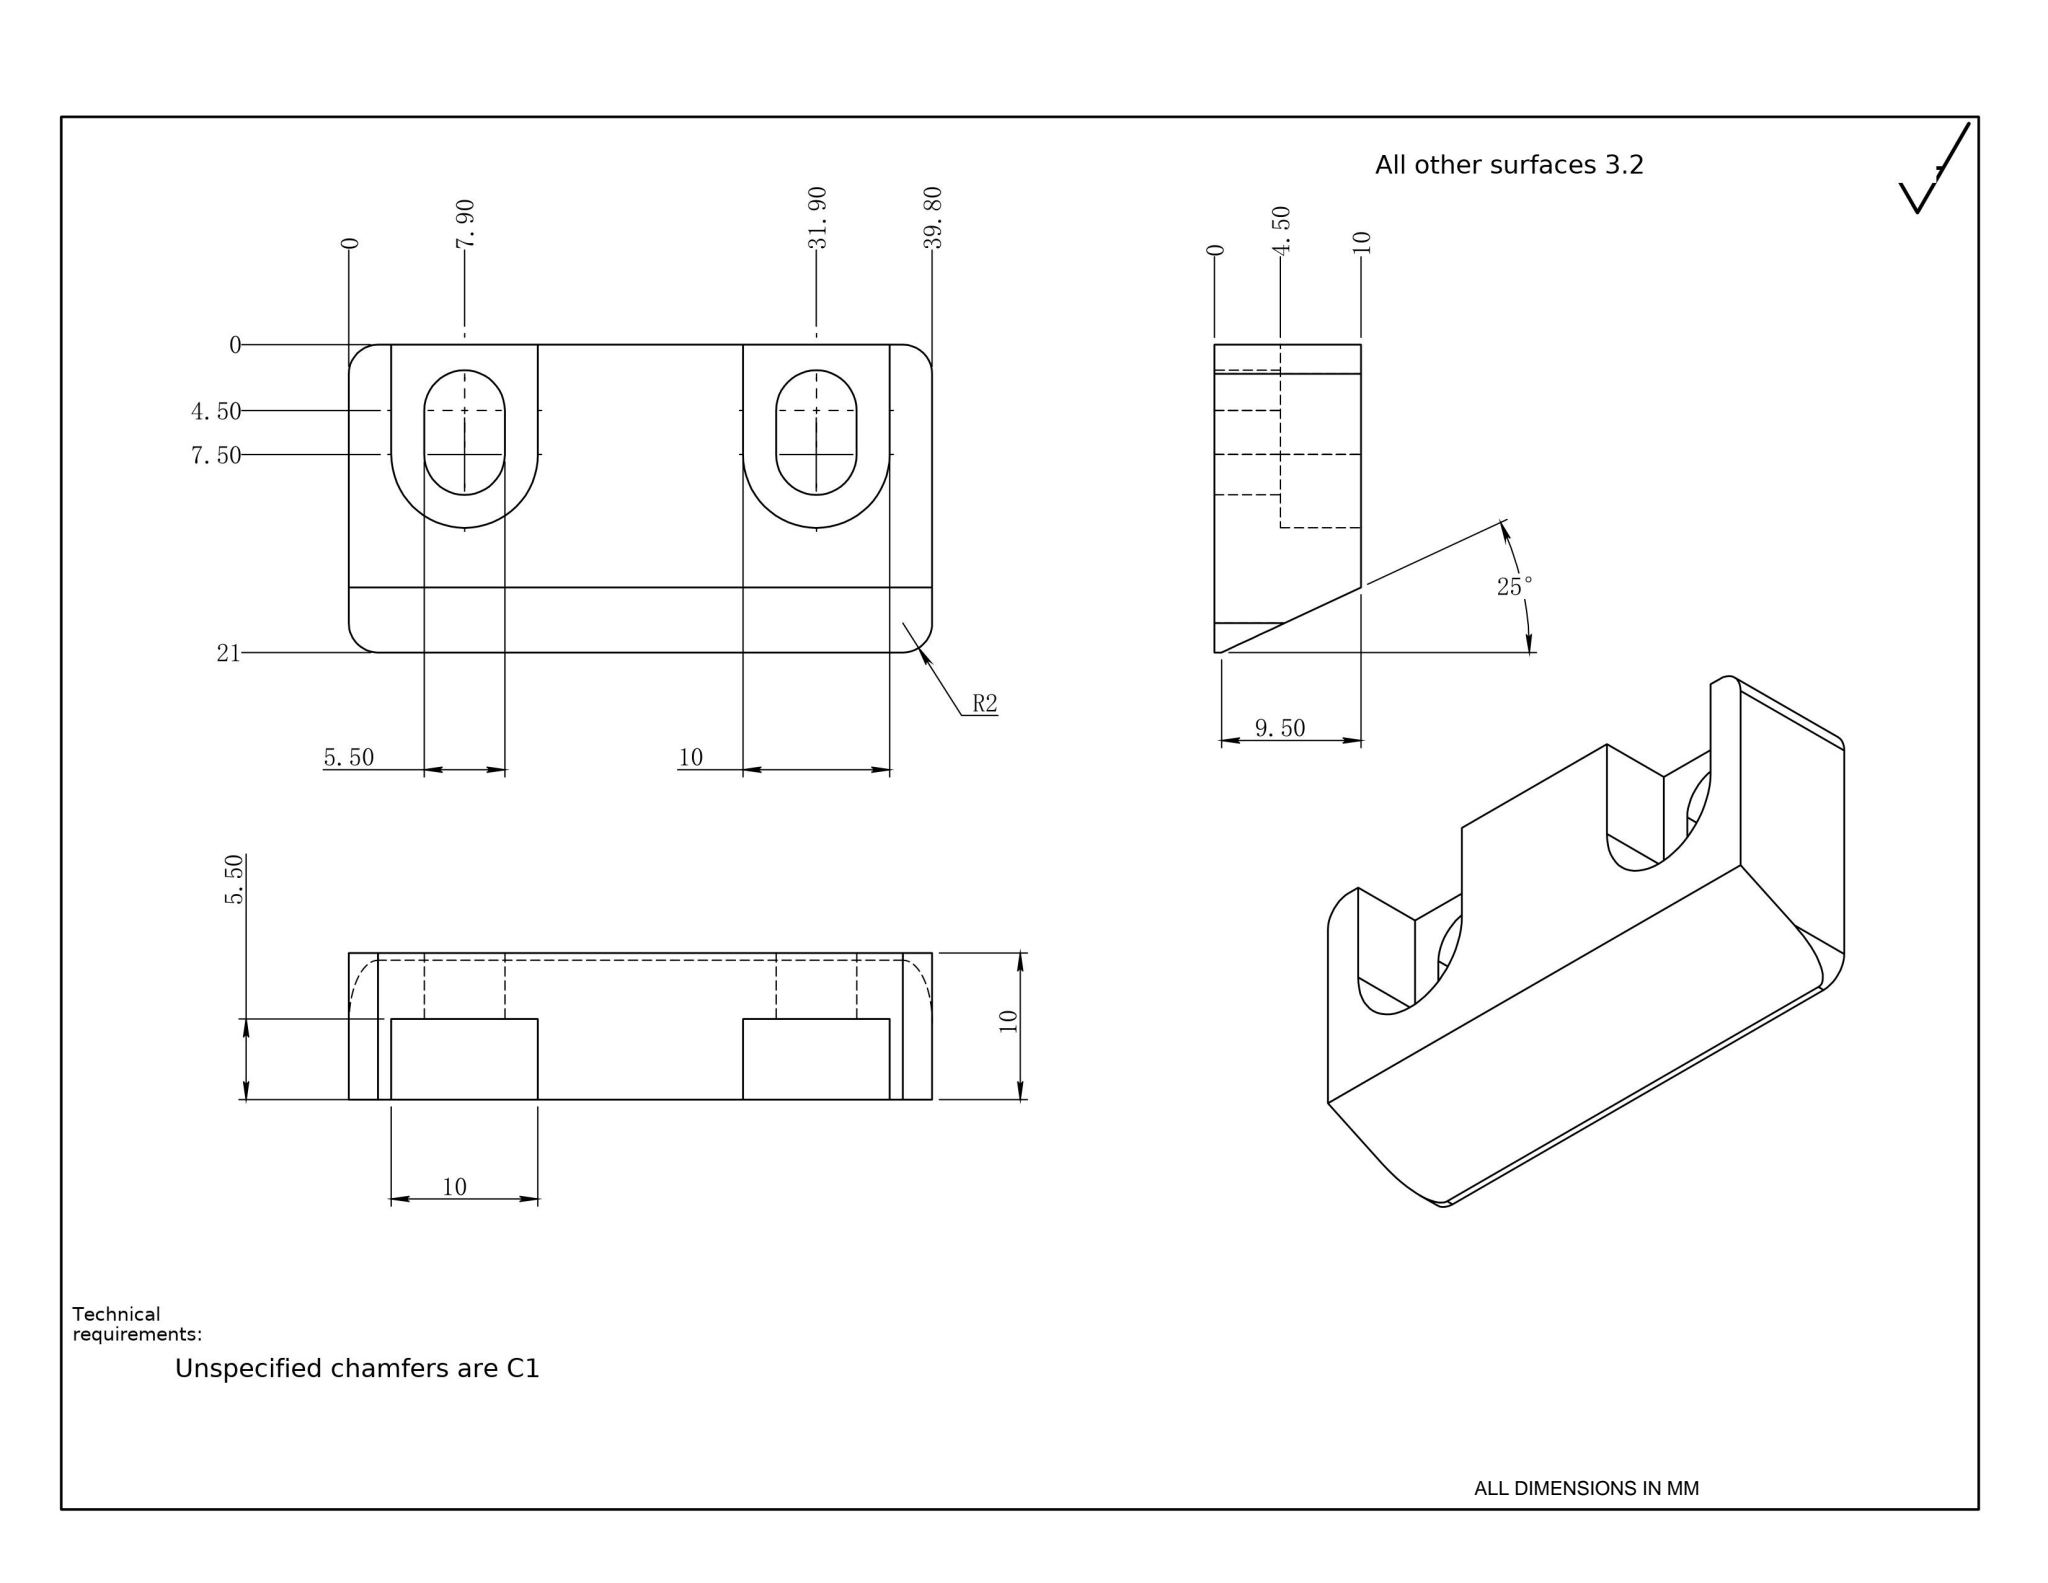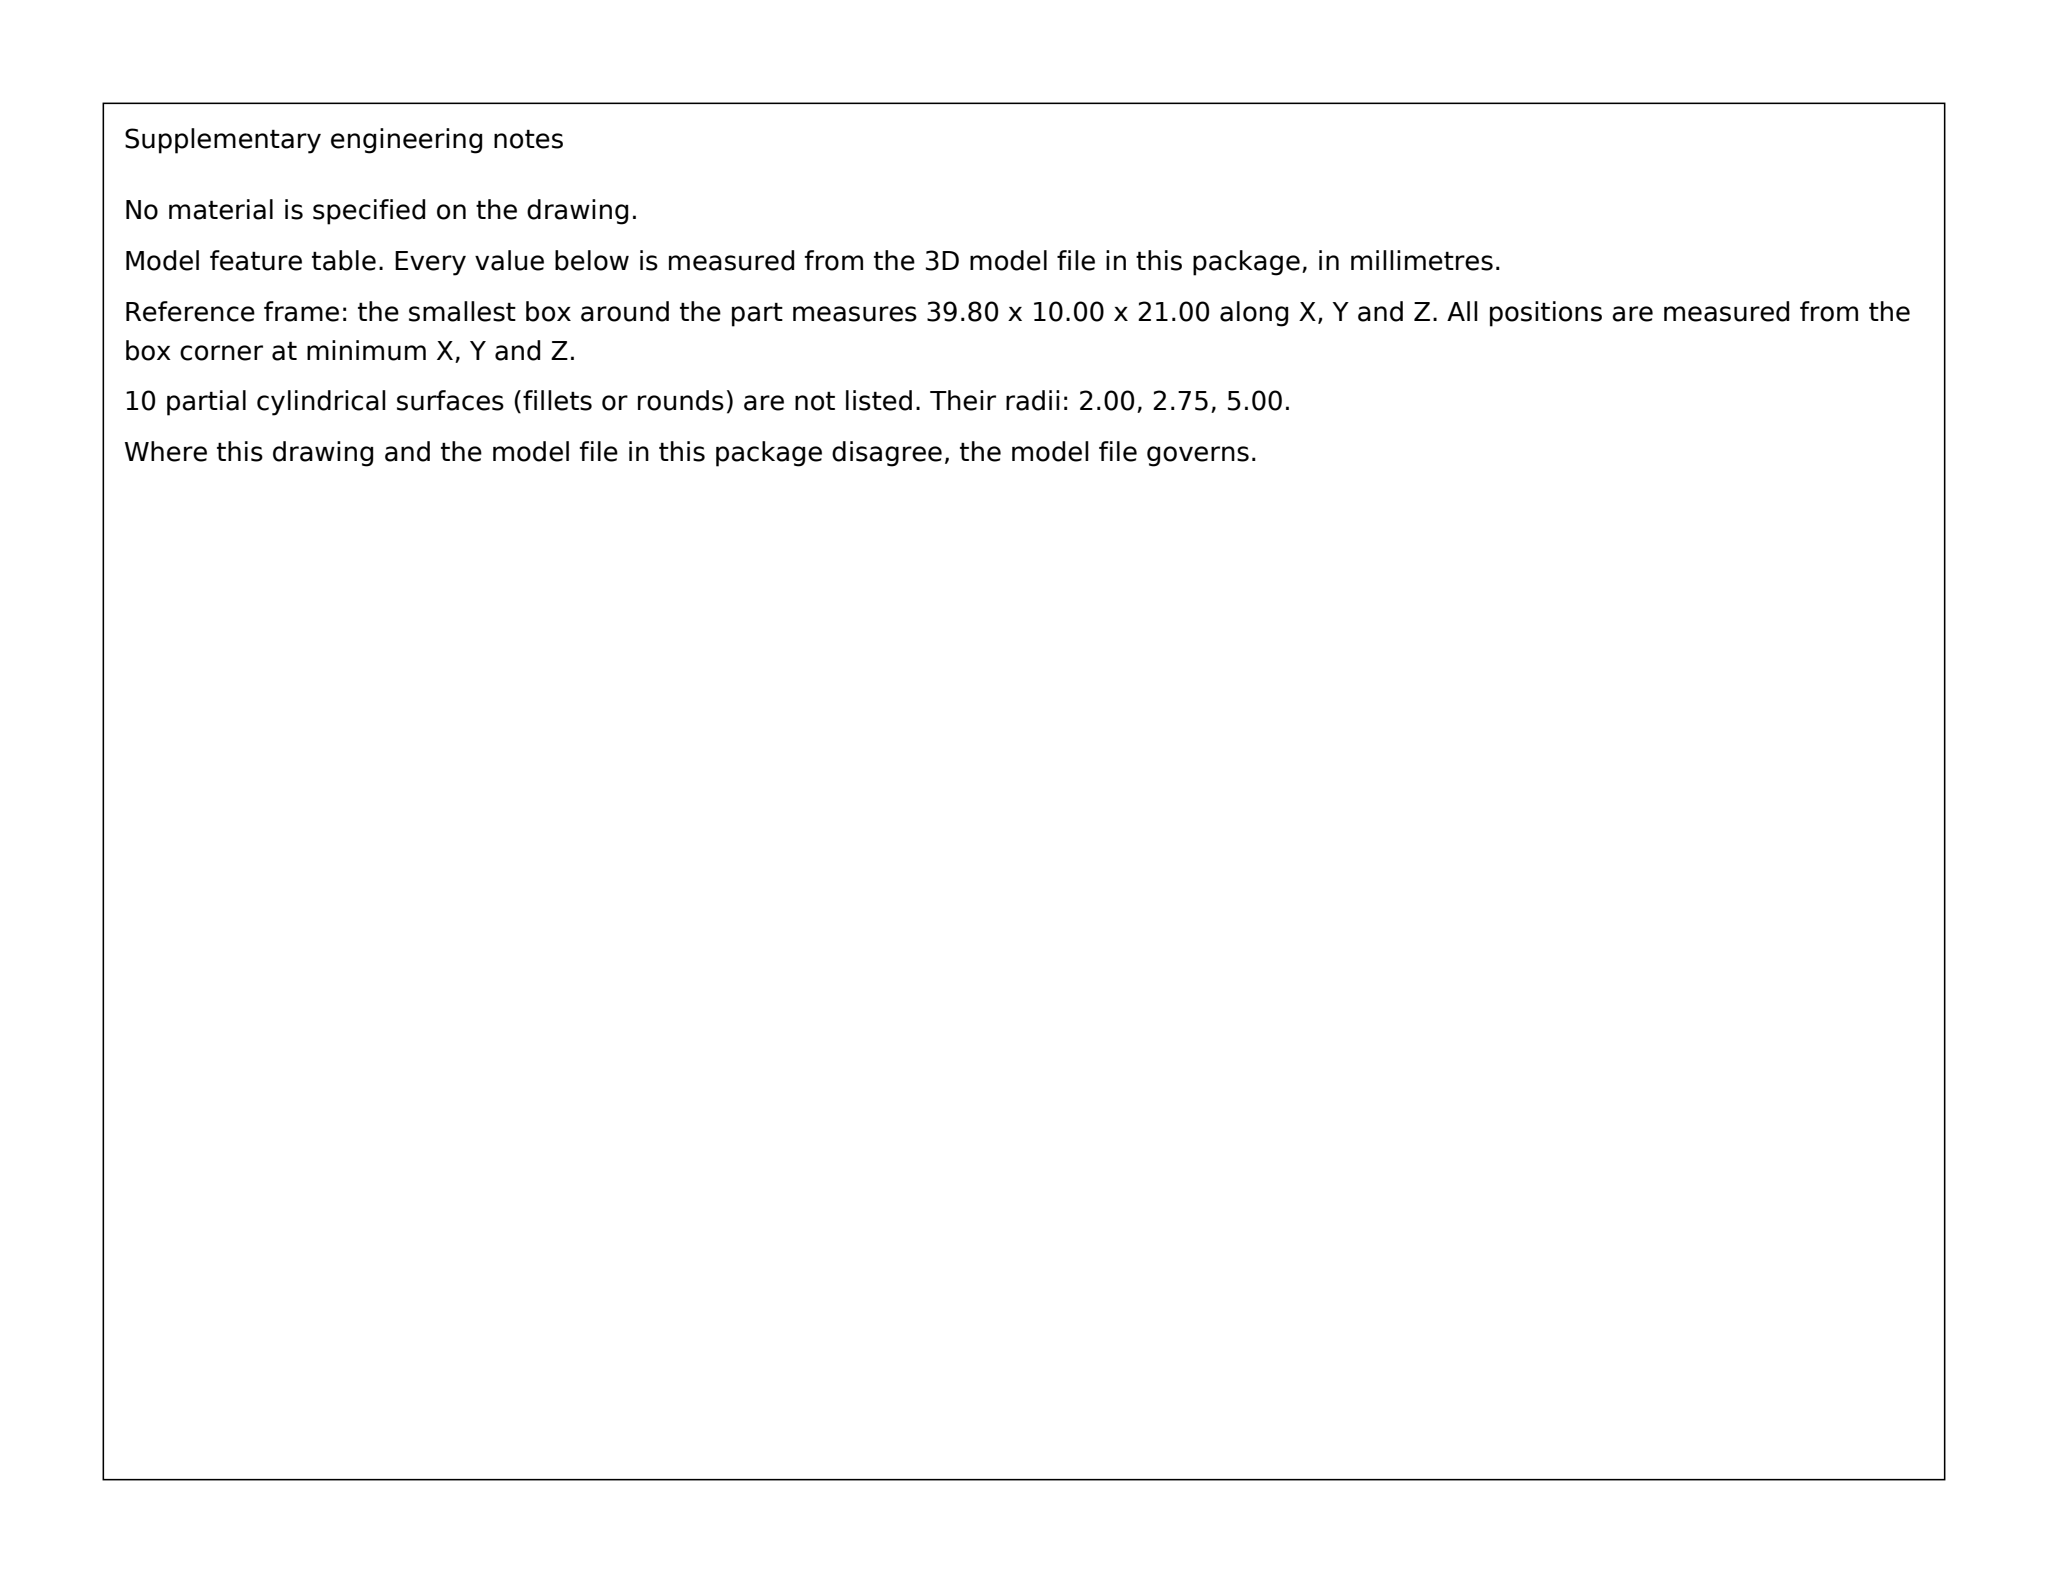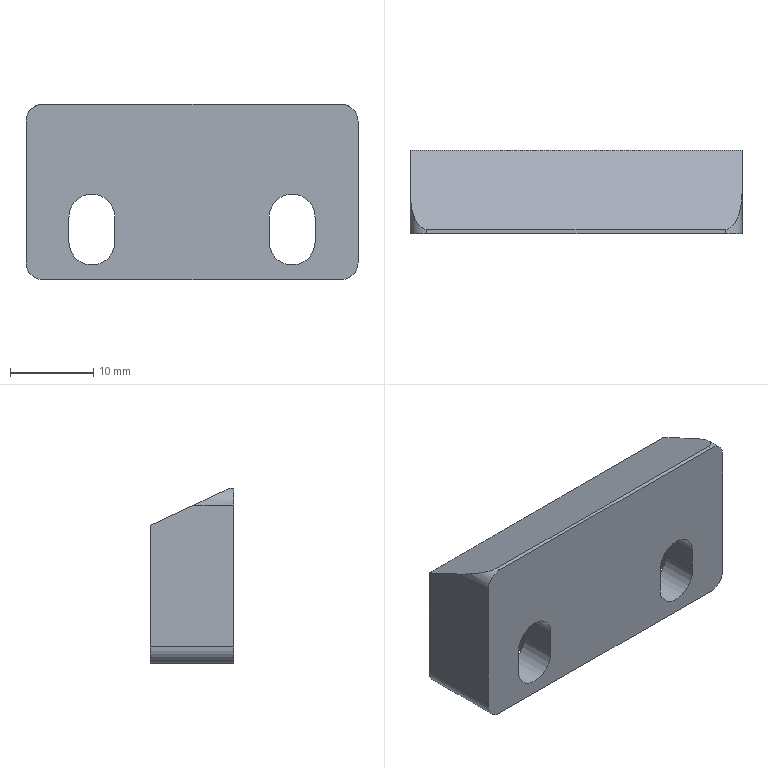Part | SolidWorks | mm | 1 solid | 31 faces | box 39.8 x 10 x 21 mm | volume 5882 mm3 | plane 17 | cylinder 14 | commonest cylinder face diameters 5.5 x6 10 x4 4 x4